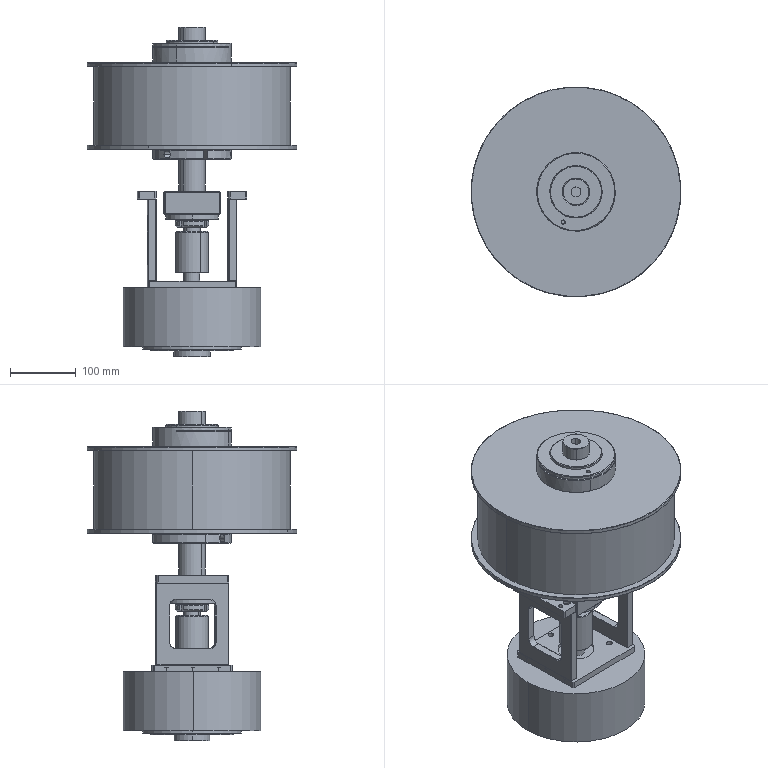Assembly | SolidWorks | mm | 20 component files | 20 solids | 683 faces | box 320 x 320 x 502 mm | volume 13999926 mm3 | cylinder 289 | plane 230 | cone 164 | commonest cylinder face diameters 5 x38 6.6 x36 11 x30 6.8 x20 3.3 x16 4.5 x16 7 x12 35 x10
Bill of materials:
8TC-A17001-20-01BearingHousing | 1 | #45 | Square block with a large stepped central through-bore and four through-holes, one near each corner.
8TC-A17001-20-02HangingShaft | 1 | #45 | Stepped cylindrical shaft or tube with three diameters, getting smaller toward one end, and a small axial bore.
8TC-A17001-20-03LocatingPlate | 1 | 6061 Alloy | Thick disc with a central bore and a radial slit from the bore to the outer edge (split-collar form). A second radial slot on the opposite side stops short of the rim. It has several axial and radial holes.
8TC-A17001-20-04Baffle1 | 1 | Tempered Glass | Thin flat circular plate with a small central hole and four small holes in a square or circular pattern around it.
8TC-A17001-20-05Baffle2 | 1 | Tempered Glass | Thin flat circular plate (annulus) with a medium-to-large central opening and four very small holes spaced around it.
8TC-A17001-20-06CoreSleeve | 1 | #45 | Thick-walled cylindrical sleeve with a central through-bore and three small radial holes in a line along one side.
8TC-A17001-20-07LockingSleeve | 1 | #45 | Thick ring with a large central bore, a partial circumferential slot cut through the wall near one face, and one small axial hole.
8TC-A17001-20-08BearingCap | 1 | A3 | Flat annular flange ring with three through-holes equally spaced and a step or chamfer at the inner bore edge.
8TC-A17001-20-09MountingPlate1 | 2 | A3 | Rectangular bar or plate with chamfered corners and six through-holes in two rows of three. One row appears counterbored or larger on the top face.
8TC-A17001-20-10MountingPlate2 | 2 | A3 | Square frame plate with a large rounded-square central window and three small holes in one narrow edge face.
8TC-A17001-20-11MountingPlate | 1 | A3 | Square flat plate with chamfered corners, a large central through-hole, and nine smaller through-holes around it (six small and three larger).
DeepGrooveBallBearing6007 | 1 | A3 | Plain thick annular ring with a central bore, square outer edges, and a fine circular line on one face.
GB812RoundNutM35_1.5 | 2 | A3 | Thin flat annular ring with a large central bore. Rectangular slots are cut through the full thickness at the outer rim. Outer edges are chamfered on both faces. The shape is similar to a slotted round nut or lock ring.
GL-56x64-15-25LightCoupling | 1 |  | Plain hollow cylindrical sleeve. It is longer than its outer diameter, has a concentric through bore, and has small chamfers on the end edges.
HB-114BHysteresisClutch | 1 | A3 | Large short cylindrical body. On one face, a smaller cylindrical shaft sticks out from a low circular boss and has an elongated slot along its length. Three small holes sit on that face. The opposite face has thin stepped circular bosses and a central hub. The overall form is similar to a simplified motor-style housing with an output shaft.
One-wayBearing6207 | 1 | A3 | Thick flat annular ring with a plain central bore and straight cylindrical outer and inner surfaces. A thin concentric line near the outer edge and another near the bore on one face suggest a separate inner and outer ring, so the shape may be a simplified bearing-style ring.
Mates:
1. coincident | 8TC-A17001-20-10MountingPlate2-3 face at (671.537, 199.71, 30.814) dir (0, 0, 1) | 8TC-A17001-20-09MountingPlate1-3 face at (664.038, 199.587, 30.814) dir (0, 0, -1)
2. coincident | 8TC-A17001-20-10MountingPlate2-3 face at (678.441, 144.816, -94.186) dir (0.9999, 0.01645, 0) | 8TC-A17001-20-09MountingPlate1-3 face at (678.441, 144.816, 30.814) dir (0.9999, 0.01645, 0)
3. width | 8TC-A17001-20-10MountingPlate2-3 face at (676.631, 254.801, -94.186) dir (-0.01645, 0.9999, 0) | 8TC-A17001-20-10MountingPlate2-3 face at (678.441, 144.816, -94.186) dir (0.01645, -0.9999, 0) | 8TC-A17001-20-09MountingPlate1-3 face at (678.441, 144.816, 30.814) dir (0.01645, -0.9999, 0) | 8TC-A17001-20-09MountingPlate1-3 face at (676.631, 254.801, 30.814) dir (-0.01645, 0.9999, 0)
4. coincident | 8TC-A17001-20-10MountingPlate2-2 face at (794.52, 201.734, 30.5) dir (0, 0, 1) | 8TC-A17001-20-09MountingPlate1-2 face at (802.019, 201.857, 30.5) dir (0, 0, -1)
5. coincident | 8TC-A17001-20-10MountingPlate2-2 face at (787.616, 256.627, -94.5) dir (-0.9999, -0.01645, 0) | 8TC-A17001-20-09MountingPlate1-2 face at (787.616, 256.627, 30.5) dir (-0.9999, -0.01645, 0)
6. width | 8TC-A17001-20-09MountingPlate1-2 face at (787.616, 256.627, 30.5) dir (-0.01645, 0.9999, 0) | 8TC-A17001-20-09MountingPlate1-2 face at (789.426, 146.642, 30.5) dir (0.01645, -0.9999, 0) | 8TC-A17001-20-10MountingPlate2-2 face at (787.616, 256.627, -94.5) dir (-0.01645, 0.9999, 0) | 8TC-A17001-20-10MountingPlate2-2 face at (789.426, 146.642, -94.5) dir (0.01645, -0.9999, 0)
7. concentric | 8TC-A17001-20-10MountingPlate2-2 face at (793.862, 241.728, -94.5) dir (0, 0, -1) r 2.5 | 8TC-A17001-20-11MountingPlate-1 face at (793.862, 241.728, -104.5) dir (0, 0, -1) r 3.3
8. concentric | 8TC-A17001-20-10MountingPlate2-2 face at (794.52, 201.734, -94.5) dir (0, 0, -1) r 2.5 | 8TC-A17001-20-11MountingPlate-1 face at (794.52, 201.734, -104.5) dir (0, 0, -1) r 3.3
9. coincident | 8TC-A17001-20-10MountingPlate2-2 face at (794.52, 201.734, -94.5) dir (0, 0, -1) | 8TC-A17001-20-11MountingPlate-1 face at (733.029, 200.722, -94.5) dir (0, 0, 1)
10. concentric | 8TC-A17001-20-11MountingPlate-1 face at (732.157, 253.715, -94.5) dir (0, 0, 1) r 4.5 | HB-114BHysteresisClutch-1 face at (732.157, 253.715, -104.5) dir (0, 0, 1) r 3.4
11. coincident | 8TC-A17001-20-11MountingPlate-1 face at (733.029, 200.722, -104.5) dir (0, 0, -1) | HB-114BHysteresisClutch-1 face at (731.301, 305.708, -104.5) dir (0, 0, 1)
12. coincident | 8TC-A17001-20-03LocatingPlate-1 face at (733.029, 200.722, 106.5) dir (0, 0, 1) | 8TC-A17001-20-04Baffle1-1 face at (733.029, 200.722, 106.5) dir (0, 0, -1)
13. distance | 8TC-A17001-20-03LocatingPlate-1 face at (733.029, 200.722, 91.5) dir (0, 0, -1) | 8TC-A17001-20-01BearingHousing-1 face at (733.029, 200.722, 42.5) dir (0, 0, 1)
14. concentric | 8TC-A17001-20-03LocatingPlate-1 face at (733.029, 200.722, 91.5) dir (0, 0, 1) r 20 | 8TC-A17001-20-02HangingShaft-1 face at (733.029, 200.722, -47.5) dir (0, 0, -1) r 20
15. concentric | 8TC-A17001-20-03LocatingPlate-1 face at (755.788, 250.792, 106.5) dir (0, 0, 1) r 1.65 | 8TC-A17001-20-04Baffle1-1 face at (755.788, 250.792, 112.5) dir (0, 0, 1) r 2.25
16. coincident | 8TC-A17001-20-04Baffle1-1 face at (733.029, 200.722, 112.5) dir (0, 0, 1) | 8TC-A17001-20-06CoreSleeve-1 face at (733.029, 200.722, 112.5) dir (0, 0, -1)
17. distance | 8TC-A17001-20-04Baffle1-1 face at (733.029, 200.722, 112.5) dir (0, 0, 1) | 8TC-A17001-20-05Baffle2-1 face at (733.029, 200.722, 232.5) dir (0, 0, -1)
18. concentric | 8TC-A17001-20-04Baffle1-1 face at (733.029, 200.722, 112.5) dir (0, 0, -1) r 20.25 | 8TC-A17001-20-02HangingShaft-1 face at (733.029, 200.722, -47.5) dir (0, 0, -1) r 20
19. concentric | 8TC-A17001-20-01BearingHousing-1 face at (733.029, 200.722, 21.5) dir (0, 0, -1) r 31 | DeepGrooveBallBearing6007-1 face at (733.029, 200.722, 14.5) dir (0, 0, -1) r 31
20. coincident | 8TC-A17001-20-01BearingHousing-1 face at (733.029, 200.722, 21.5) dir (0, 0, -1) | DeepGrooveBallBearing6007-1 face at (732.519, 231.718, 21.5) dir (0, 0, 1)
21. coincident | 8TC-A17001-20-01BearingHousing-1 face at (733.029, 200.722, 25.5) dir (0, 0, 1) | One-wayBearing6207-1 face at (733.029, 200.722, 25.5) dir (0, 0, -1)
22. concentric | 8TC-A17001-20-01BearingHousing-1 face at (733.029, 200.722, 25.5) dir (0, 0, 1) r 36 | One-wayBearing6207-1 face at (733.029, 200.722, 42.5) dir (0, 0, -1) r 36
23. coincident | 8TC-A17001-20-01BearingHousing-1 face at (733.029, 200.722, 7.5) dir (0, 0, -1) | 8TC-A17001-20-08BearingCap-1 face at (733.029, 200.722, 7.5) dir (0, 0, 1)
24. concentric | 8TC-A17001-20-01BearingHousing-1 face at (751.025, 170.703, 7.5) dir (0, 0, -1) r 2.5 | 8TC-A17001-20-08BearingCap-1 face at (751.025, 170.703, -0.5) dir (0, 0, -1) r 3.3
25. concentric | DeepGrooveBallBearing6007-1 face at (733.029, 200.722, 14.5) dir (0, 0, -1) r 17.5 | 8TC-A17001-20-02HangingShaft-1 face at (733.029, 200.722, -47.5) dir (0, 0, -1) r 17.5
26. coincident | DeepGrooveBallBearing6007-1 face at (732.675, 222.219, 7.5) dir (0, 0, -1) | GB812RoundNutM35_1.5-1 face at (733.029, 200.722, 7.5) dir (0, 0, 1)
27. concentric | 8TC-A17001-20-05Baffle2-1 face at (733.029, 200.722, 238.5) dir (0, 0, -1) r 40.25 | 8TC-A17001-20-06CoreSleeve-1 face at (733.029, 200.722, 112.5) dir (0, 0, 1) r 39.75
28. concentric | 8TC-A17001-20-07LockingSleeve-1 face at (686.739, 181.82, 238.5) dir (0, 0, -1) r 1.65 | 8TC-A17001-20-05Baffle2-1 face at (686.739, 181.82, 232.5) dir (0, 0, -1) r 2.25
29. coincident | 8TC-A17001-20-07LockingSleeve-1 face at (733.029, 200.722, 238.5) dir (0, 0, -1) | 8TC-A17001-20-05Baffle2-1 face at (733.029, 200.722, 238.5) dir (0, 0, 1)
30. concentric | 8TC-A17001-20-06CoreSleeve-1 face at (733.029, 200.722, 112.5) dir (0, 0, 1) r 39.75 | 8TC-A17001-20-02HangingShaft-1 face at (733.029, 200.722, -47.5) dir (0, 0, -1) r 20
31. concentric | 8TC-A17001-20-07LockingSleeve-1 face at (733.029, 200.722, 268.5) dir (0, 0, -1) r 40 | 8TC-A17001-20-06CoreSleeve-1 face at (733.029, 200.722, 112.5) dir (0, 0, 1) r 39.75
32. concentric | 8TC-A17001-20-02HangingShaft-1 face at (733.029, 200.722, -47.5) dir (0, 0, -1) r 17.5 | 8TC-A17001-20-08BearingCap-1 face at (733.029, 200.722, 7.5) dir (0, 0, -1) r 40
33. concentric | 8TC-A17001-20-02HangingShaft-1 face at (733.029, 200.722, -47.5) dir (0, 0, -1) r 17.5 | GB812RoundNutM35_1.5-1 face at (733.029, 200.722, -2.5) dir (0, 0, 1) r 17.5
34. concentric | 8TC-A17001-20-02HangingShaft-1 face at (733.029, 200.722, -47.5) dir (0, 0, -1) r 17.5 | GB812RoundNutM35_1.5-2 face at (733.029, 200.722, -2.5) dir (0, 0, -1) r 17.5
35. coincident | GB812RoundNutM35_1.5-1 face at (733.029, 200.722, -2.5) dir (0, 0, -1) | GB812RoundNutM35_1.5-2 face at (733.029, 200.722, -2.5) dir (0, 0, 1)
36. coincident | 8TC-A17001-20-04Baffle1-1 face at (733.029, 200.722, 112.5) dir (0, 0, 1) | MaximumCoilSize-1 face at (733.029, 200.722, 112.5) dir (0, 0, -1)
37. coincident | 8TC-A17001-20-01BearingHousing-1 face at (733.029, 200.722, 42.5) dir (0, 0, 1) | 8TC-A17001-20-09MountingPlate1-2 face at (802.019, 201.857, 42.5) dir (0, 0, 1)
38. concentric | 8TC-A17001-20-06CoreSleeve-1 face at (733.029, 200.722, 112.5) dir (0, 0, 1) r 39.75 | MaximumCoilSize-1 face at (733.029, 200.722, 232.5) dir (0, 0, -1) r 150
39. concentric | 8TC-A17001-20-02HangingShaft-1 face at (733.029, 200.722, -47.5) dir (0, 0, -1) r 12.5 | GL-56x64-15-25LightCoupling-1 face at (733.029, 200.722, -18.5) dir (0, 0, -1) r 25
40. concentric | 8TC-A17001-20-02HangingShaft-1 face at (733.029, 200.722, -47.5) dir (0, 0, -1) r 12.5 | HB-114BHysteresisClutch-1 face at (733.029, 200.722, -58.5) dir (0, 0, -1) r 12.5